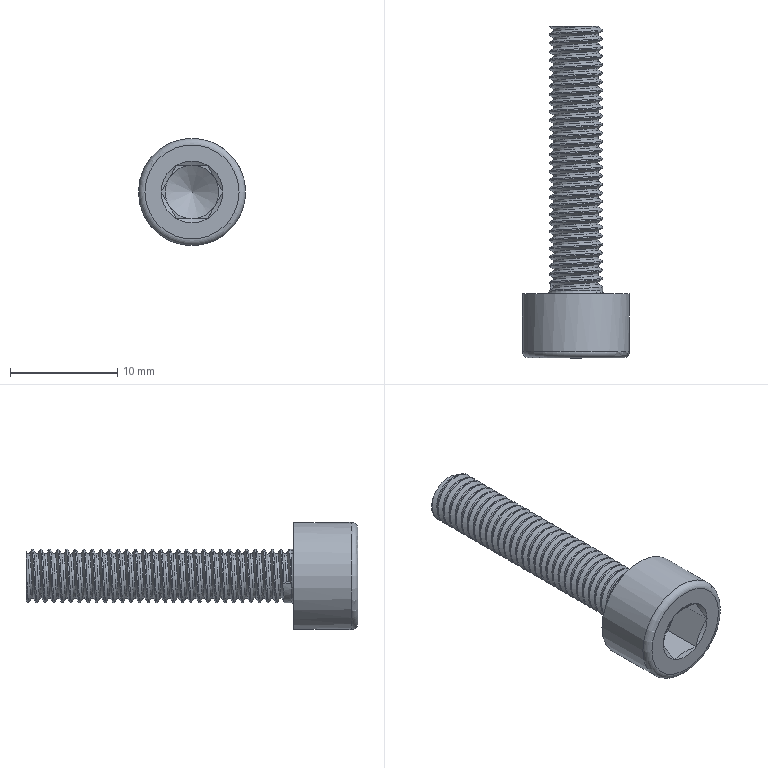Component | NX | M5X25_HEX_BOLT_2 | 1 solid | 30 faces | volume 779 mm3 | plane 16 | cone 7 | cylinder 3 | torus 2 | spline 2 | commonest cylinder face diameters 5 x1 10 x1 4.2 x1